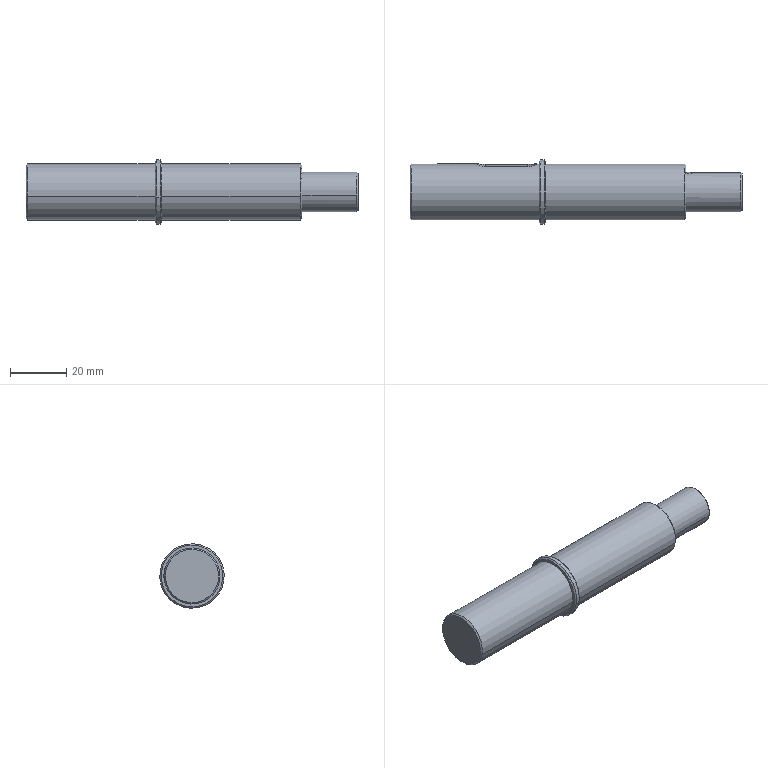Component | SolidWorks | ChainPartDriveShaft-1 | 1 solid | 31 faces | box 118.3 x 23 x 23 mm | volume 33570 mm3 | cylinder 11 | plane 11 | cone 9 | commonest cylinder face diameters 20 x4 23 x2 14 x2 6 x2 4 x1
build123d program:
from build123d import *

# Parameters (mm, degrees)
CUT_EXTRUDE1_DEPTH = 3.5
CHAMFER1_SIZE      = 0.5
CUT_EXTRUDE2_DEPTH = 2.5


with BuildPart() as part:
    # Sketch1 → Revolve1 (revolve)
    with BuildSketch(Plane.XY, mode=Mode.PRIVATE) as revolve1_sk:
        Polygon((0, 0), (7, 0), (7, 20), (10, 20), (10, 70), (11.5, 70), (11.5, 72.3), (10, 72.3), (10, 118.3), (0, 118.3), align=None)
    revolve(revolve1_sk.sketch.rotate(Axis((0, 0, 0), (0, 1, 0)), 90), axis=Axis((0, 0, 0), (0, 1, 0)))

    # Sketch2 → Cut-Extrude1 (cut)
    with BuildSketch(Plane.XY.offset(10)):
        with BuildLine():
            Line((3, 91.3), (3, 76.3))
            ThreePointArc((3, 76.3), (0, 73.3), (-3, 76.3))
            Line((-3, 76.3), (-3, 91.3))
            ThreePointArc((-3, 91.3), (0, 94.3), (3, 91.3))
        make_face()
    extrude(amount=-CUT_EXTRUDE1_DEPTH, mode=Mode.SUBTRACT)

    # Chamfer1
    chamfer1_edges = [part.edges().sort_by_distance(p)[0] for p in [
        (0, 0, 7),
        (0, 118.3, 10),
        (0, 72.3, 11.5),
        (0, 70, 11.5),
        (0, 20, 10),
    ]]
    chamfer(chamfer1_edges, length=CHAMFER1_SIZE)

    # Sketch3 → Cut-Extrude2 (cut)
    with BuildSketch(Plane.XY.offset(7)):
        with BuildLine():
            Line((2, 18), (2, 0))
            ThreePointArc((2, 0), (0, -2), (-2, 0))
            Line((-2, 0), (-2, 18))
            ThreePointArc((-2, 18), (0, 20), (2, 18))
        make_face()
    extrude(amount=-CUT_EXTRUDE2_DEPTH, mode=Mode.SUBTRACT)


solid = part.part

# Placed as in the assembly
solid = solid.moved(Location((198.637, -2.563, -35.304), (-80.909, 0, 90)))